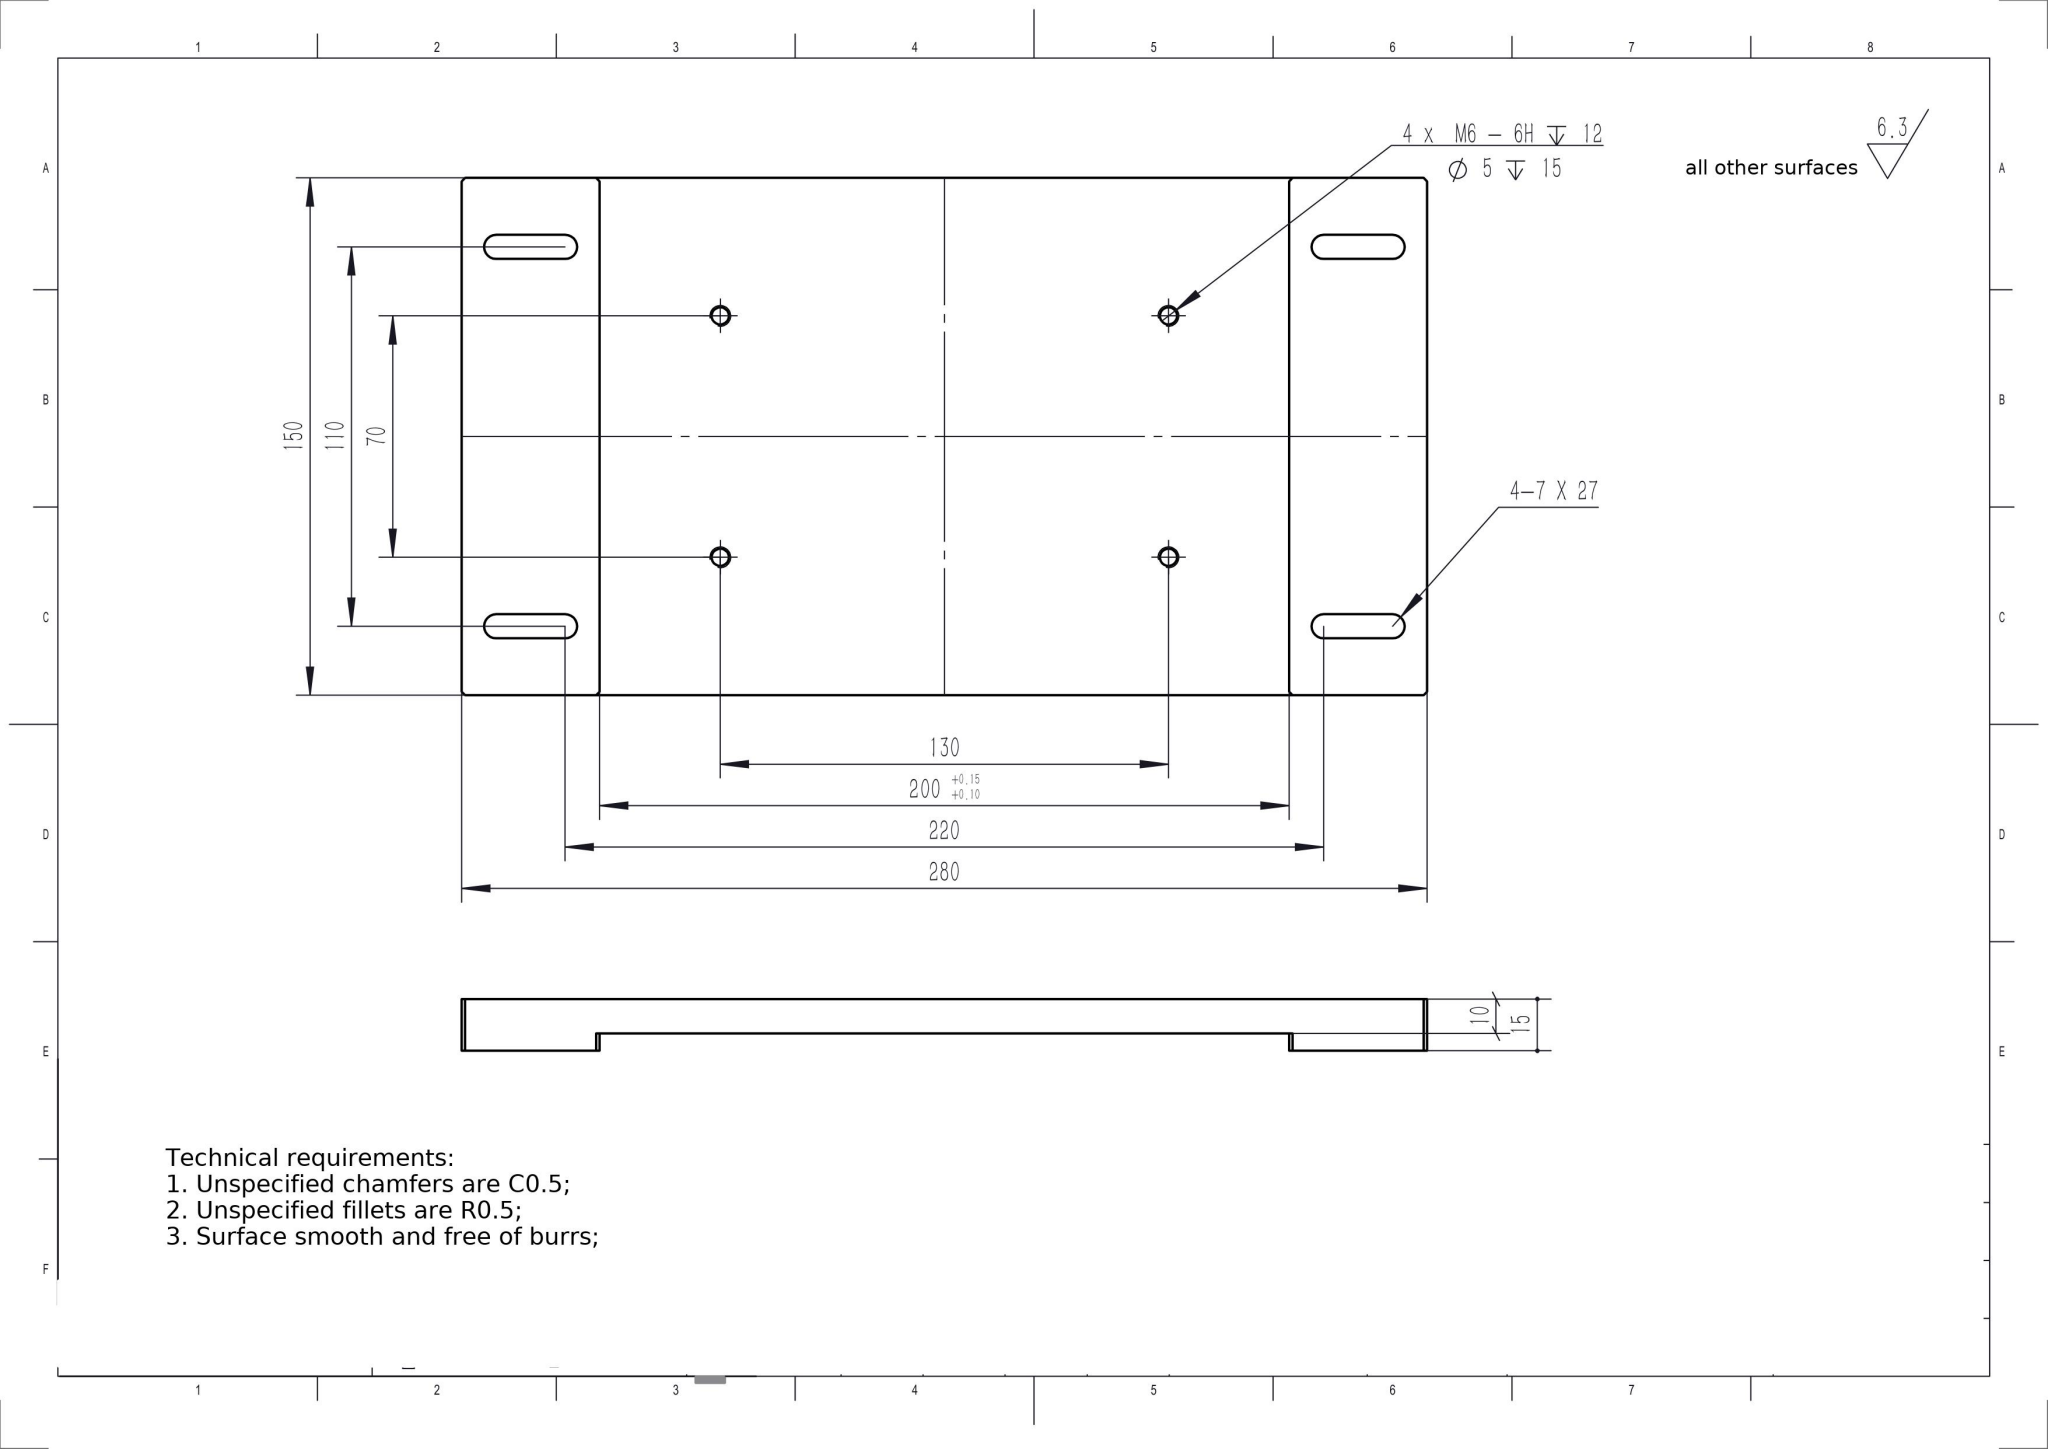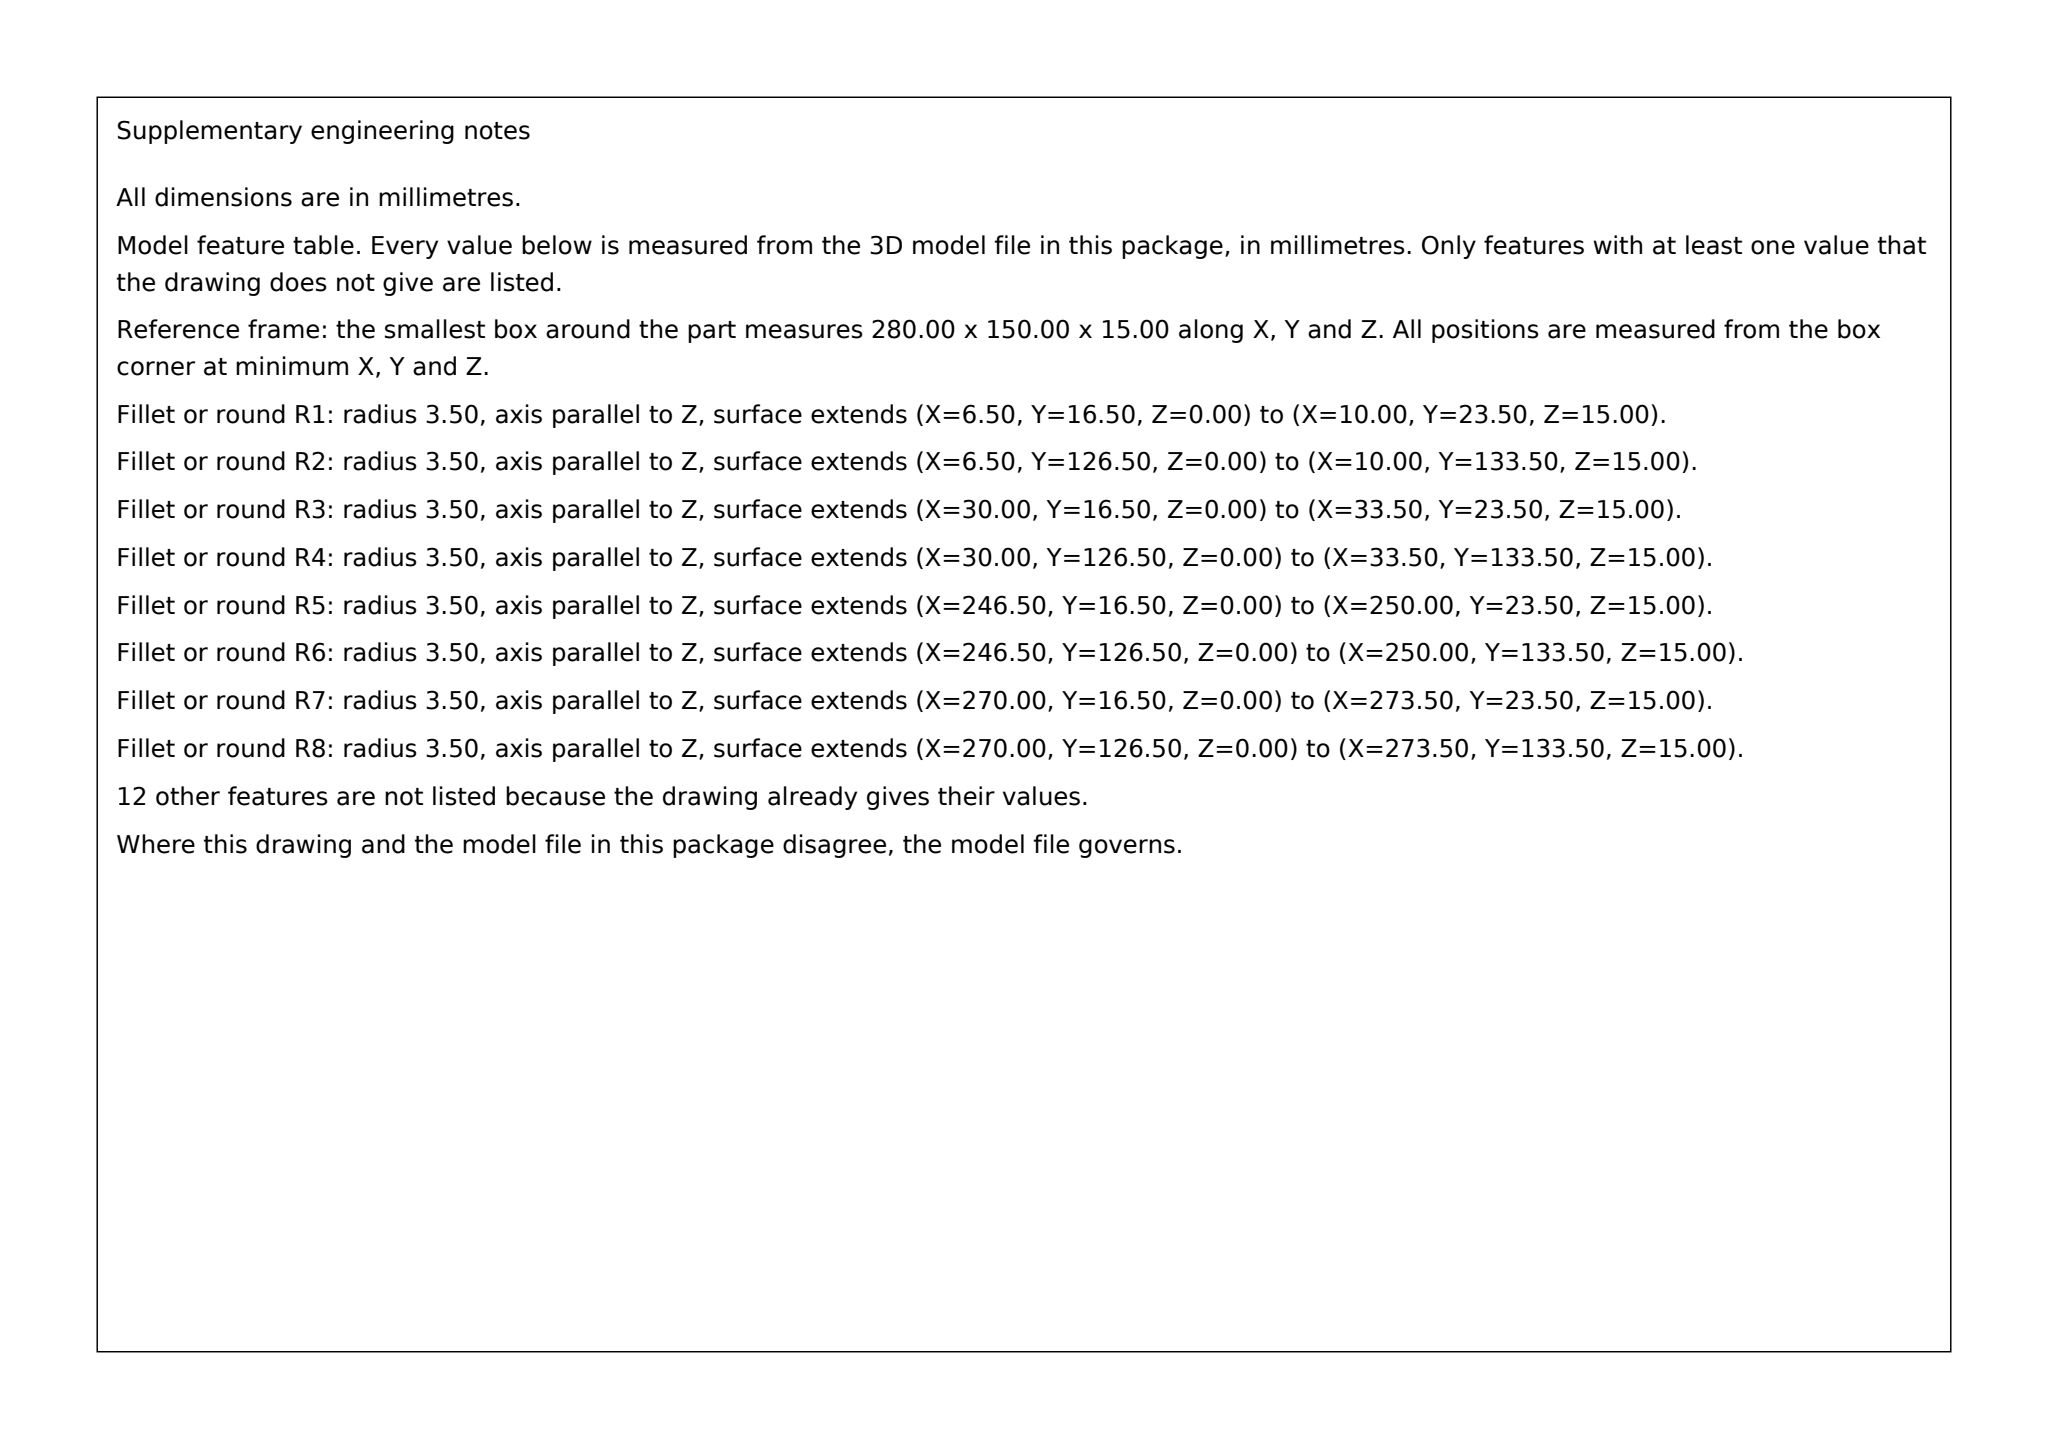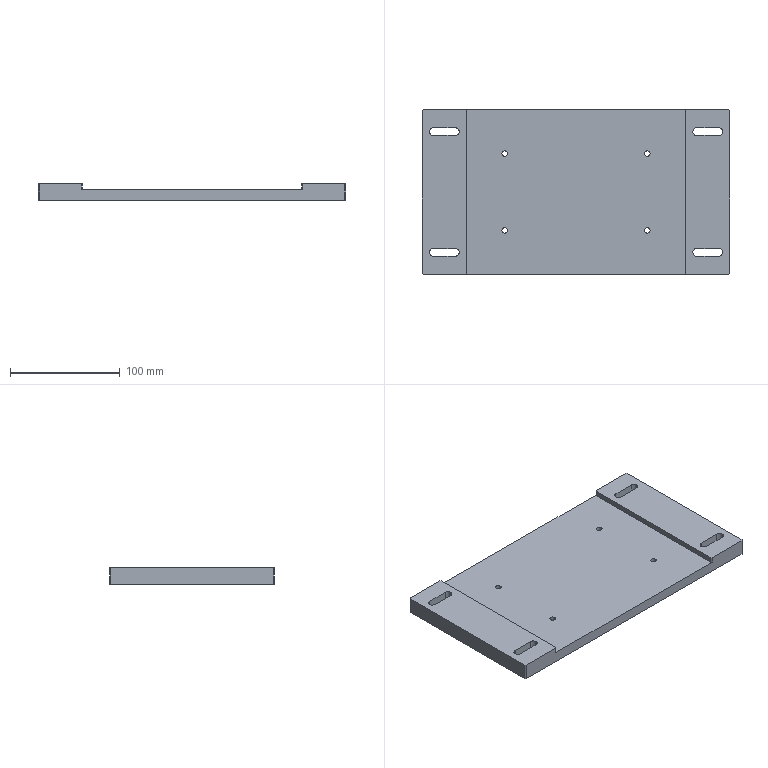Part | SolidWorks | mm | 1 solid | 46 faces | box 280 x 150 x 15 mm | volume 468466 mm3 | plane 26 | cylinder 20 | commonest cylinder face diameters 7 x12 5 x8
build123d program:
from build123d import *

# Parameters (mm, degrees)
SKETCH1_W             = 280
SKETCH1_H             = 150
BOSS_EXTRUDE1_DEPTH   = 15
SKETCH2_W             = 200
SKETCH2_H             = 150
CUT_EXTRUDE1_DEPTH    = 5
CUT_EXTRUDE2_DEPTH    = 160.531
M6_TAPPED_HOLE1_D     = 5
M6_TAPPED_HOLE1_DEPTH = 15
M6_TAPPED_HOLE1_TIP   = 1.502
CHAMFER1_SIZE         = 1


with BuildPart() as part:
    # Sketch1 → Boss-Extrude1 (new body)
    with BuildSketch(Plane.XY):
        Rectangle(SKETCH1_W, SKETCH1_H)
    extrude(amount=BOSS_EXTRUDE1_DEPTH)

    # Sketch2 → Cut-Extrude1 (cut)
    with BuildSketch(Plane.XY.offset(15)):
        Rectangle(SKETCH2_W, SKETCH2_H)
    extrude(amount=-CUT_EXTRUDE1_DEPTH, mode=Mode.SUBTRACT)

    # Sketch3 → Cut-Extrude2 (cut, through all)
    with BuildSketch(Plane.XY.offset(15)):
        with BuildLine():
            Line((-130, 58.5), (-110, 58.5))
            ThreePointArc((-110, 58.5), (-106.5, 55), (-110, 51.5))
            Line((-110, 51.5), (-130, 51.5))
            ThreePointArc((-130, 51.5), (-133.5, 55), (-130, 58.5))
        make_face()
        with BuildLine():
            Line((-130, -58.5), (-110, -58.5))
            ThreePointArc((-110, -58.5), (-106.5, -55), (-110, -51.5))
            Line((-110, -51.5), (-130, -51.5))
            ThreePointArc((-130, -51.5), (-133.5, -55), (-130, -58.5))
        make_face()
        with BuildLine():
            Line((130, 58.5), (110, 58.5))
            ThreePointArc((110, 58.5), (106.5, 55), (110, 51.5))
            Line((110, 51.5), (130, 51.5))
            ThreePointArc((130, 51.5), (133.5, 55), (130, 58.5))
        make_face()
        with BuildLine():
            Line((130, -58.5), (110, -58.5))
            ThreePointArc((110, -58.5), (106.5, -55), (110, -51.5))
            Line((110, -51.5), (130, -51.5))
            ThreePointArc((130, -51.5), (133.5, -55), (130, -58.5))
        make_face()
    extrude(amount=-CUT_EXTRUDE2_DEPTH, mode=Mode.SUBTRACT)

    # M6 Tapped Hole1
    with Locations(Plane.XY.offset(10)):
        with Locations((-65, 35), (-65, -35), (65, -35), (65, 35)):
            Hole(M6_TAPPED_HOLE1_D / 2, depth=M6_TAPPED_HOLE1_DEPTH)
            with Locations((0, 0, -(M6_TAPPED_HOLE1_DEPTH + M6_TAPPED_HOLE1_TIP / 2))):  # 118° drill point
                Cone(0, M6_TAPPED_HOLE1_D / 2, M6_TAPPED_HOLE1_TIP, mode=Mode.SUBTRACT)

    # Chamfer1
    chamfer1_edges = [part.edges().sort_by_distance(p)[0] for p in [
        (100, 75, 12.5),
        (100, -75, 12.5),
        (-100, -75, 12.5),
        (-100, 75, 12.5),
        (140, -75, 7.5),
        (-140, -75, 7.5),
        (-140, 75, 7.5),
        (140, 75, 7.5),
    ]]
    chamfer(chamfer1_edges, length=CHAMFER1_SIZE)


solid = part.part